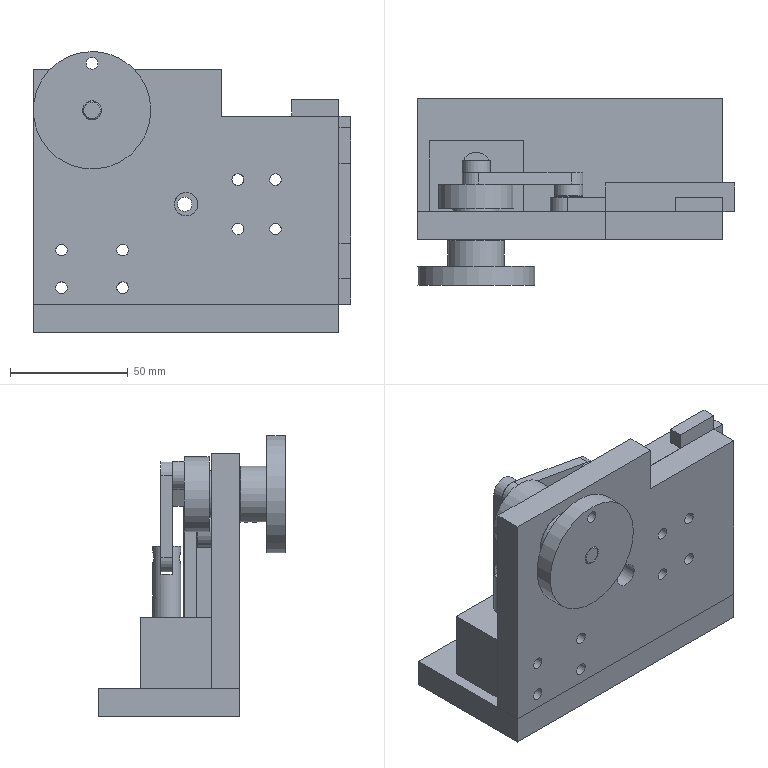Assembly | NX | mm | 13 component files | 13 solids | 180 faces | box 135 x 79.5 x 119.5 mm | volume 356067 mm3 | plane 111 | cylinder 64 | cone 5 | commonest cylinder face diameters 5 x20 12 x9 5.5 x8 10 x7 5.1 x6 6.1 x2 8 x2 15 x2
Bill of materials:
unnamed part 1 | 1 |  | Rectangular plate with a stepped profile: a thinner back web with raised pads/ribs on one face separated by two recesses, plus four through holes in a 2x2 pattern.
unnamed part 2 | 1 |  | Thin flat plate of uniform thickness. One long edge is straight; the opposite edge has two V-shaped notches, giving a sawtooth-like profile.
unnamed part 3 | 1 |  | Flanged disc with a cylindrical boss on one side. It has a central through bore and one smaller off-center through hole in the flange.
unnamed part 4 | 1 |  | Rectangular block with one large through hole along one axis and four smaller through holes in a rectangular pattern along a perpendicular axis.
unnamed part 5 | 1 |  | Stepped cylindrical shaft with a large disc-shaped head, a thin collar, a middle-diameter step, and a smaller chamfered end. It has one small off-center through hole in the head.
unnamed part 6 | 2 |  | Flat bar of uniform thickness with one fully rounded end containing a single through hole. The opposite end is cut to a symmetric pointed V tip.
unnamed part 7 | 1 |  | Solid cylindrical pin with an open slot across one end, forming two tines, and a cross hole through both tines perpendicular to the slot. The other end is plain and flat.
unnamed part 8 | 1 |  | Flat rectangular plate with one larger through hole and two smaller through holes near one long edge.
unnamed part 9 | 1 |  | Thin elongated strap with one rounded end and one square end. Along its length it has a round hole near the rounded end, an elongated slot, a second round hole, and an open U-shaped slot at the square end.
unnamed part 10 | 1 |  | Flat plate of uniform thickness with a rectangular step cut from one corner. It has one large hole, one medium central hole, and two groups of four small holes in rectangular patterns.
unnamed part 11 | 1 |  | Flat link with two fully rounded ends, each with a through hole. One hole is visibly larger than the other.
unnamed part 12 | 1 |  | Flat link with fully rounded ends and two equal-size through holes, one at each end.
Mates:
1. touch align | groove_guide_block 1 face | upright_plate 1 face
2. touch align | groove_guide_block 1 edge | upright_plate 1 edge
3. concentric | groove_guide_block 1 edge | upright_plate 1 edge
4. fix | upright_plate 1 component
5. concentric | short_link 1 edge | slider_rod 1 edge
6. fix | round_guide_block 1 component
7. parallel | long_link 1 face | bi_link 1 face
8. concentric | long_link 1 edge | bi_link 1 edge
9. fix | eccentric_cam 1 component
10. concentric | long_link 1 edge | eccentric_cam 1 edge
11. touch align | hand_wheel 1 face | eccentric_cam 1 face
12. concentric | eccentric_cam 1 edge | hand_wheel 1 edge
13. fix | bi_link 1 component
14. distance | tri_slider 2 face | bi_link 1 face
15. touch align | tri_slider 2 face | groove_guide_block 1 face
16. touch align | upright_plate 1 face | V_slider 1 face
17. touch align | V_slider 1 face | groove_guide_block 1 face
18. fix | tri_slider 1 component
19. distance | V_slider 1 face | groove_guide_block 1 face